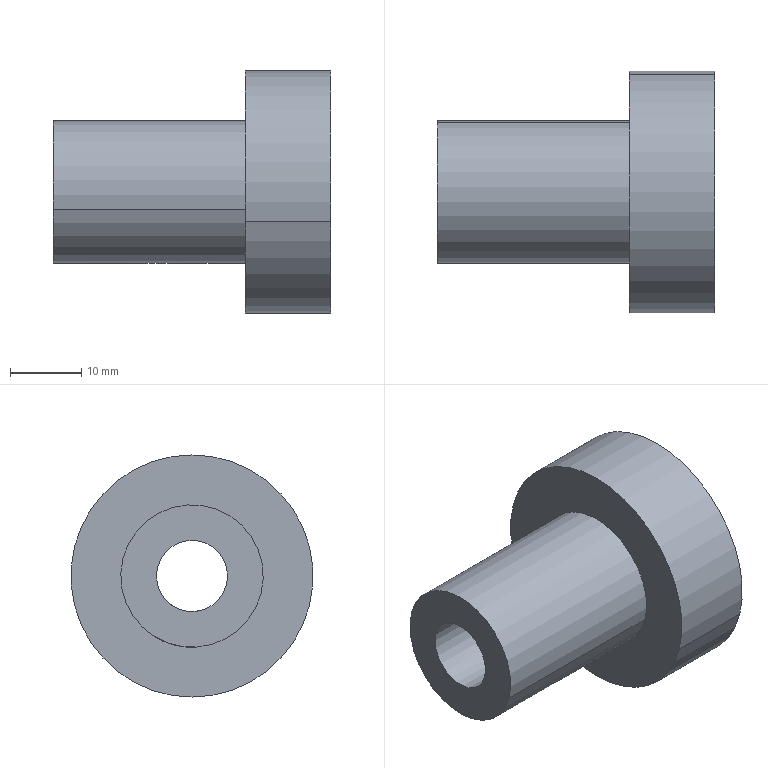Component | SolidWorks | MiddleAxisUpperSleeve-1 | 1 solid | 21 faces | box 39 x 34 x 34 mm | volume 14393 mm3 | cylinder 12 | plane 5 | cone 4 | commonest cylinder face diameters 3.2 x2 17 x2 30 x2 34 x2 20 x2 10 x2 | material 5154-O, Bar (SS)
STEP:
#1=COLOUR_RGB('',0.7922,0.8196,0.9333);
#2=FILL_AREA_STYLE_COLOUR('',#1);
#3=FILL_AREA_STYLE('',(#2));
#4=SURFACE_STYLE_FILL_AREA(#3);
#5=SURFACE_SIDE_STYLE('',(#4));
#6=SURFACE_STYLE_USAGE(.BOTH.,#5);
#7=PRESENTATION_STYLE_ASSIGNMENT((#6));
#8=CARTESIAN_POINT('',(5.711,0.7019,13.575));
#9=VERTEX_POINT('',#8);
#10=CARTESIAN_POINT('',(5.711,0.5797,13.544));
#11=VERTEX_POINT('',#10);
#12=CARTESIAN_POINT('',(5.711,0.7019,13.575));
#13=CARTESIAN_POINT('',(5.719,0.7019,13.575));
#14=CARTESIAN_POINT('',(5.728,0.7004,13.574));
#15=CARTESIAN_POINT('',(5.739,0.6962,13.571));
#16=CARTESIAN_POINT('',(5.743,0.6944,13.57));
#17=CARTESIAN_POINT('',(5.75,0.6903,13.568));
#18=CARTESIAN_POINT('',(5.753,0.6879,13.567));
#19=CARTESIAN_POINT('',(5.761,0.68,13.562));
#20=CARTESIAN_POINT('',(5.766,0.6736,13.559));
#21=CARTESIAN_POINT('',(5.771,0.6628,13.555));
#22=CARTESIAN_POINT('',(5.772,0.6591,13.554));
#23=CARTESIAN_POINT('',(5.774,0.6514,13.551));
#24=CARTESIAN_POINT('',(5.774,0.6474,13.55));
#25=CARTESIAN_POINT('',(5.774,0.6393,13.548));
#26=CARTESIAN_POINT('',(5.774,0.6353,13.547));
#27=CARTESIAN_POINT('',(5.772,0.6273,13.546));
#28=CARTESIAN_POINT('',(5.771,0.6233,13.545));
#29=CARTESIAN_POINT('',(5.766,0.6119,13.544));
#30=CARTESIAN_POINT('',(5.761,0.6048,13.543));
#31=CARTESIAN_POINT('',(5.753,0.596,13.543));
#32=CARTESIAN_POINT('',(5.75,0.5932,13.543));
#33=CARTESIAN_POINT('',(5.743,0.5885,13.543));
#34=CARTESIAN_POINT('',(5.739,0.5865,13.543));
#35=CARTESIAN_POINT('',(5.732,0.5832,13.544));
#36=CARTESIAN_POINT('',(5.728,0.5819,13.544));
#37=CARTESIAN_POINT('',(5.719,0.5802,13.544));
#38=CARTESIAN_POINT('',(5.715,0.5797,13.544));
#39=CARTESIAN_POINT('',(5.711,0.5797,13.544));
#40=B_SPLINE_CURVE_WITH_KNOTS('',3,(#12,#13,#14,#15,#16,#17,#18,#19,#20,#21,#22,#23,#24,#25,#26,#27,#28,#29,#30,#31,#32,#33,#34,#35,#36,#37,#38,#39),.UNSPECIFIED.,.F.,.F.,(4,2,2,2,2,2,2,2,2,2,2,2,2,4),(0.005036,0.005665,0.005979,0.006294,0.006923,0.007238,0.007553,0.007867,0.008182,0.008811,0.009126,0.00944,0.009755,0.01007),.UNSPECIFIED.);
#41=EDGE_CURVE('',#9,#11,#40,.T.);
#42=ORIENTED_EDGE('',*,*,#41,.F.);
#43=CARTESIAN_POINT('',(5.711,0.7372,13.435));
#44=VERTEX_POINT('',#43);
#45=CARTESIAN_POINT('',(5.711,0.7527,13.374));
#46=DIRECTION('',(0.,0.2451,-0.9695));
#47=VECTOR('',#46,39.37);
#48=LINE('',#45,#47);
#49=EDGE_CURVE('',#9,#44,#48,.T.);
#50=ORIENTED_EDGE('',*,*,#49,.T.);
#51=CARTESIAN_POINT('',(5.711,0.6151,13.404));
#52=VERTEX_POINT('',#51);
#53=CARTESIAN_POINT('',(5.711,0.6762,13.42));
#54=DIRECTION('',(0.,0.2451,-0.9695));
#55=DIRECTION('',(0.,-0.9695,-0.2451));
#56=AXIS2_PLACEMENT_3D('',#53,#54,#55);
#57=CIRCLE('',#56,0.06299);
#58=EDGE_CURVE('',#44,#52,#57,.T.);
#59=ORIENTED_EDGE('',*,*,#58,.T.);
#60=CARTESIAN_POINT('',(5.711,0.6305,13.343));
#61=DIRECTION('',(0.,0.2451,-0.9695));
#62=VECTOR('',#61,39.37);
#63=LINE('',#60,#62);
#64=EDGE_CURVE('',#11,#52,#63,.T.);
#65=ORIENTED_EDGE('',*,*,#64,.F.);
#66=EDGE_LOOP('',(#42,#50,#59,#65));
#67=FACE_OUTER_BOUND('',#66,.T.);
#68=CARTESIAN_POINT('',(5.711,0.6916,13.358));
#69=DIRECTION('',(0.,0.2451,-0.9695));
#70=DIRECTION('',(0.,-0.9695,-0.2451));
#71=AXIS2_PLACEMENT_3D('',#68,#69,#70);
#72=CYLINDRICAL_SURFACE('',#71,0.06299);
#73=ADVANCED_FACE('',(#67),#72,.F.);
#74=ORIENTED_EDGE('',*,*,#58,.F.);
#75=CARTESIAN_POINT('',(5.711,0.7946,13.401));
#76=VERTEX_POINT('',#75);
#77=CARTESIAN_POINT('',(5.711,0.8137,13.389));
#78=DIRECTION('',(-0.,0.8589,-0.5122));
#79=VECTOR('',#78,39.37);
#80=LINE('',#77,#79);
#81=EDGE_CURVE('',#44,#76,#80,.T.);
#82=ORIENTED_EDGE('',*,*,#81,.T.);
#83=CARTESIAN_POINT('',(5.711,0.5809,13.347));
#84=VERTEX_POINT('',#83);
#85=CARTESIAN_POINT('',(5.711,0.5809,13.347));
#86=CARTESIAN_POINT('',(5.727,0.5809,13.347));
#87=CARTESIAN_POINT('',(5.742,0.5836,13.347));
#88=CARTESIAN_POINT('',(5.764,0.5913,13.346));
#89=CARTESIAN_POINT('',(5.771,0.5945,13.346));
#90=CARTESIAN_POINT('',(5.785,0.6022,13.347));
#91=CARTESIAN_POINT('',(5.791,0.6066,13.347));
#92=CARTESIAN_POINT('',(5.803,0.6165,13.347));
#93=CARTESIAN_POINT('',(5.808,0.622,13.347));
#94=CARTESIAN_POINT('',(5.818,0.6341,13.348));
#95=CARTESIAN_POINT('',(5.823,0.6406,13.349));
#96=CARTESIAN_POINT('',(5.83,0.6543,13.351));
#97=CARTESIAN_POINT('',(5.832,0.6616,13.352));
#98=CARTESIAN_POINT('',(5.836,0.6764,13.355));
#99=CARTESIAN_POINT('',(5.837,0.6838,13.357));
#100=CARTESIAN_POINT('',(5.837,0.6991,13.36));
#101=CARTESIAN_POINT('',(5.836,0.7065,13.362));
#102=CARTESIAN_POINT('',(5.832,0.7209,13.367));
#103=CARTESIAN_POINT('',(5.83,0.7279,13.369));
#104=CARTESIAN_POINT('',(5.823,0.7408,13.374));
#105=CARTESIAN_POINT('',(5.818,0.7469,13.377));
#106=CARTESIAN_POINT('',(5.808,0.7581,13.382));
#107=CARTESIAN_POINT('',(5.803,0.7631,13.384));
#108=CARTESIAN_POINT('',(5.785,0.7766,13.391));
#109=CARTESIAN_POINT('',(5.771,0.7833,13.394));
#110=CARTESIAN_POINT('',(5.749,0.7901,13.398));
#111=CARTESIAN_POINT('',(5.742,0.7918,13.399));
#112=CARTESIAN_POINT('',(5.727,0.794,13.4));
#113=CARTESIAN_POINT('',(5.719,0.7946,13.401));
#114=CARTESIAN_POINT('',(5.711,0.7946,13.401));
#115=B_SPLINE_CURVE_WITH_KNOTS('',3,(#85,#86,#87,#88,#89,#90,#91,#92,#93,#94,#95,#96,#97,#98,#99,#100,#101,#102,#103,#104,#105,#106,#107,#108,#109,#110,#111,#112,#113,#114),.UNSPECIFIED.,.F.,.F.,(4,2,2,2,2,2,2,2,2,2,2,2,2,2,4),(0.01171,0.01289,0.01348,0.01406,0.01465,0.01524,0.01583,0.01642,0.017,0.01759,0.01818,0.01877,0.01994,0.02053,0.02112),.UNSPECIFIED.);
#116=EDGE_CURVE('',#84,#76,#115,.T.);
#117=ORIENTED_EDGE('',*,*,#116,.F.);
#118=CARTESIAN_POINT('',(5.711,0.5695,13.328));
#119=DIRECTION('',(0.,-0.5122,-0.8589));
#120=VECTOR('',#119,39.37);
#121=LINE('',#118,#120);
#122=EDGE_CURVE('',#52,#84,#121,.T.);
#123=ORIENTED_EDGE('',*,*,#122,.F.);
#124=EDGE_LOOP('',(#74,#82,#117,#123));
#125=FACE_OUTER_BOUND('',#124,.T.);
#126=CARTESIAN_POINT('',(5.711,0.6916,13.358));
#127=DIRECTION('',(0.,0.2451,-0.9695));
#128=DIRECTION('',(0.,-0.9695,-0.2451));
#129=AXIS2_PLACEMENT_3D('',#126,#127,#128);
#130=CONICAL_SURFACE('',#129,0.126,0.7854);
#131=ADVANCED_FACE('',(#125),#130,.F.);
#132=CARTESIAN_POINT('',(6.42,0.9195,13.822));
#133=VERTEX_POINT('',#132);
#134=CARTESIAN_POINT('',(6.42,0.2707,13.658));
#135=VERTEX_POINT('',#134);
#136=CARTESIAN_POINT('',(6.42,0.5951,13.74));
#137=DIRECTION('',(1.,0.,0.));
#138=DIRECTION('',(0.,-0.9695,-0.2451));
#139=AXIS2_PLACEMENT_3D('',#136,#137,#138);
#140=CIRCLE('',#139,0.3346);
#141=EDGE_CURVE('',#133,#135,#140,.T.);
#142=ORIENTED_EDGE('',*,*,#141,.F.);
#143=CARTESIAN_POINT('',(6.577,0.9195,13.822));
#144=VERTEX_POINT('',#143);
#145=CARTESIAN_POINT('',(9.528,0.9195,13.822));
#146=DIRECTION('',(1.,0.,0.));
#147=VECTOR('',#146,39.37);
#148=LINE('',#145,#147);
#149=EDGE_CURVE('',#133,#144,#148,.T.);
#150=ORIENTED_EDGE('',*,*,#149,.T.);
#151=CARTESIAN_POINT('',(6.577,0.2707,13.658));
#152=VERTEX_POINT('',#151);
#153=CARTESIAN_POINT('',(6.577,0.5951,13.74));
#154=DIRECTION('',(1.,0.,0.));
#155=DIRECTION('',(0.,-0.9695,-0.2451));
#156=AXIS2_PLACEMENT_3D('',#153,#154,#155);
#157=CIRCLE('',#156,0.3346);
#158=EDGE_CURVE('',#144,#152,#157,.T.);
#159=ORIENTED_EDGE('',*,*,#158,.T.);
#160=CARTESIAN_POINT('',(9.528,0.2707,13.658));
#161=DIRECTION('',(1.,0.,0.));
#162=VECTOR('',#161,39.37);
#163=LINE('',#160,#162);
#164=EDGE_CURVE('',#135,#152,#163,.T.);
#165=ORIENTED_EDGE('',*,*,#164,.F.);
#166=EDGE_LOOP('',(#142,#150,#159,#165));
#167=FACE_OUTER_BOUND('',#166,.T.);
#168=CARTESIAN_POINT('',(9.528,0.5951,13.74));
#169=DIRECTION('',(1.,0.,0.));
#170=DIRECTION('',(0.,-0.9695,-0.2451));
#171=AXIS2_PLACEMENT_3D('',#168,#169,#170);
#172=CYLINDRICAL_SURFACE('',#171,0.3346);
#173=ADVANCED_FACE('',(#167),#172,.F.);
#174=CARTESIAN_POINT('',(6.577,1.168,13.885));
#175=VERTEX_POINT('',#174);
#176=CARTESIAN_POINT('',(6.577,0.02257,13.595));
#177=VERTEX_POINT('',#176);
#178=CARTESIAN_POINT('',(6.577,0.5951,13.74));
#179=DIRECTION('',(1.,0.,0.));
#180=DIRECTION('',(0.,-0.9695,-0.2451));
#181=AXIS2_PLACEMENT_3D('',#178,#179,#180);
#182=CIRCLE('',#181,0.5906);
#183=EDGE_CURVE('',#175,#177,#182,.T.);
#184=ORIENTED_EDGE('',*,*,#183,.F.);
#185=CARTESIAN_POINT('',(6.656,1.168,13.885));
#186=VERTEX_POINT('',#185);
#187=CARTESIAN_POINT('',(9.528,1.168,13.885));
#188=DIRECTION('',(1.,0.,0.));
#189=VECTOR('',#188,39.37);
#190=LINE('',#187,#189);
#191=EDGE_CURVE('',#175,#186,#190,.T.);
#192=ORIENTED_EDGE('',*,*,#191,.T.);
#193=CARTESIAN_POINT('',(6.656,0.02257,13.595));
#194=VERTEX_POINT('',#193);
#195=CARTESIAN_POINT('',(6.656,0.5951,13.74));
#196=DIRECTION('',(1.,0.,0.));
#197=DIRECTION('',(0.,-0.9695,-0.2451));
#198=AXIS2_PLACEMENT_3D('',#195,#196,#197);
#199=CIRCLE('',#198,0.5906);
#200=EDGE_CURVE('',#186,#194,#199,.T.);
#201=ORIENTED_EDGE('',*,*,#200,.T.);
#202=CARTESIAN_POINT('',(9.528,0.02257,13.595));
#203=DIRECTION('',(1.,0.,0.));
#204=VECTOR('',#203,39.37);
#205=LINE('',#202,#204);
#206=EDGE_CURVE('',#177,#194,#205,.T.);
#207=ORIENTED_EDGE('',*,*,#206,.F.);
#208=EDGE_LOOP('',(#184,#192,#201,#207));
#209=FACE_OUTER_BOUND('',#208,.T.);
#210=CARTESIAN_POINT('',(9.528,0.5951,13.74));
#211=DIRECTION('',(1.,0.,0.));
#212=DIRECTION('',(0.,-0.9695,-0.2451));
#213=AXIS2_PLACEMENT_3D('',#210,#211,#212);
#214=CYLINDRICAL_SURFACE('',#213,0.5906);
#215=ADVANCED_FACE('',(#209),#214,.F.);
#216=CARTESIAN_POINT('',(6.184,-0.05377,13.576));
#217=VERTEX_POINT('',#216);
#218=CARTESIAN_POINT('',(6.184,1.244,13.904));
#219=VERTEX_POINT('',#218);
#220=CARTESIAN_POINT('',(6.184,0.5951,13.74));
#221=DIRECTION('',(1.,0.,0.));
#222=DIRECTION('',(0.,-0.9695,-0.2451));
#223=AXIS2_PLACEMENT_3D('',#220,#221,#222);
#224=CIRCLE('',#223,0.6693);
#225=EDGE_CURVE('',#217,#219,#224,.T.);
#226=ORIENTED_EDGE('',*,*,#225,.T.);
#227=CARTESIAN_POINT('',(6.656,1.244,13.904));
#228=VERTEX_POINT('',#227);
#229=CARTESIAN_POINT('',(9.528,1.244,13.904));
#230=DIRECTION('',(1.,0.,0.));
#231=VECTOR('',#230,39.37);
#232=LINE('',#229,#231);
#233=EDGE_CURVE('',#219,#228,#232,.T.);
#234=ORIENTED_EDGE('',*,*,#233,.T.);
#235=CARTESIAN_POINT('',(6.656,-0.05377,13.576));
#236=VERTEX_POINT('',#235);
#237=CARTESIAN_POINT('',(6.656,0.5951,13.74));
#238=DIRECTION('',(1.,0.,0.));
#239=DIRECTION('',(0.,-0.9695,-0.2451));
#240=AXIS2_PLACEMENT_3D('',#237,#238,#239);
#241=CIRCLE('',#240,0.6693);
#242=EDGE_CURVE('',#236,#228,#241,.T.);
#243=ORIENTED_EDGE('',*,*,#242,.F.);
#244=CARTESIAN_POINT('',(9.528,-0.05377,13.576));
#245=DIRECTION('',(1.,0.,0.));
#246=VECTOR('',#245,39.37);
#247=LINE('',#244,#246);
#248=EDGE_CURVE('',#217,#236,#247,.T.);
#249=ORIENTED_EDGE('',*,*,#248,.F.);
#250=EDGE_LOOP('',(#226,#234,#243,#249));
#251=FACE_OUTER_BOUND('',#250,.T.);
#252=CARTESIAN_POINT('',(9.528,0.5951,13.74));
#253=DIRECTION('',(1.,0.,0.));
#254=DIRECTION('',(0.,-0.9695,-0.2451));
#255=AXIS2_PLACEMENT_3D('',#252,#253,#254);
#256=CYLINDRICAL_SURFACE('',#255,0.6693);
#257=ADVANCED_FACE('',(#251),#256,.T.);
#258=ORIENTED_EDGE('',*,*,#116,.T.);
#259=CARTESIAN_POINT('',(5.711,0.7946,13.401));
#260=CARTESIAN_POINT('',(5.703,0.7946,13.401));
#261=CARTESIAN_POINT('',(5.696,0.794,13.4));
#262=CARTESIAN_POINT('',(5.68,0.7918,13.399));
#263=CARTESIAN_POINT('',(5.673,0.7901,13.398));
#264=CARTESIAN_POINT('',(5.658,0.7855,13.396));
#265=CARTESIAN_POINT('',(5.651,0.7827,13.394));
#266=CARTESIAN_POINT('',(5.638,0.776,13.39));
#267=CARTESIAN_POINT('',(5.631,0.7721,13.388));
#268=CARTESIAN_POINT('',(5.619,0.7631,13.384));
#269=CARTESIAN_POINT('',(5.614,0.7581,13.382));
#270=CARTESIAN_POINT('',(5.604,0.7472,13.377));
#271=CARTESIAN_POINT('',(5.6,0.7411,13.374));
#272=CARTESIAN_POINT('',(5.593,0.7282,13.37));
#273=CARTESIAN_POINT('',(5.59,0.7214,13.367));
#274=CARTESIAN_POINT('',(5.586,0.7071,13.363));
#275=CARTESIAN_POINT('',(5.585,0.6995,13.36));
#276=CARTESIAN_POINT('',(5.585,0.6845,13.357));
#277=CARTESIAN_POINT('',(5.586,0.6769,13.355));
#278=CARTESIAN_POINT('',(5.59,0.6619,13.352));
#279=CARTESIAN_POINT('',(5.592,0.6548,13.351));
#280=CARTESIAN_POINT('',(5.603,0.634,13.348));
#281=CARTESIAN_POINT('',(5.613,0.6217,13.347));
#282=CARTESIAN_POINT('',(5.631,0.6067,13.347));
#283=CARTESIAN_POINT('',(5.637,0.6023,13.347));
#284=CARTESIAN_POINT('',(5.651,0.5946,13.346));
#285=CARTESIAN_POINT('',(5.658,0.5914,13.346));
#286=CARTESIAN_POINT('',(5.673,0.5862,13.347));
#287=CARTESIAN_POINT('',(5.68,0.5842,13.347));
#288=CARTESIAN_POINT('',(5.696,0.5815,13.347));
#289=CARTESIAN_POINT('',(5.703,0.5809,13.347));
#290=CARTESIAN_POINT('',(5.711,0.5809,13.347));
#291=B_SPLINE_CURVE_WITH_KNOTS('',3,(#259,#260,#261,#262,#263,#264,#265,#266,#267,#268,#269,#270,#271,#272,#273,#274,#275,#276,#277,#278,#279,#280,#281,#282,#283,#284,#285,#286,#287,#288,#289,#290),.UNSPECIFIED.,.F.,.F.,(4,2,2,2,2,2,2,2,2,2,2,2,2,2,2,4),(0.0023,0.002888,0.003477,0.004065,0.004653,0.005242,0.00583,0.006419,0.007007,0.007595,0.008184,0.00936,0.009949,0.01054,0.01113,0.01171),.UNSPECIFIED.);
#292=EDGE_CURVE('',#76,#84,#291,.T.);
#293=ORIENTED_EDGE('',*,*,#292,.T.);
#294=EDGE_LOOP('',(#258,#293));
#295=FACE_BOUND('',#294,.T.);
#296=CARTESIAN_POINT('',(5.121,0.2134,13.644));
#297=VERTEX_POINT('',#296);
#298=CARTESIAN_POINT('',(5.121,0.9768,13.837));
#299=VERTEX_POINT('',#298);
#300=CARTESIAN_POINT('',(5.121,0.5951,13.74));
#301=DIRECTION('',(1.,0.,0.));
#302=DIRECTION('',(0.,-0.9695,-0.2451));
#303=AXIS2_PLACEMENT_3D('',#300,#301,#302);
#304=CIRCLE('',#303,0.3937);
#305=EDGE_CURVE('',#297,#299,#304,.T.);
#306=ORIENTED_EDGE('',*,*,#305,.T.);
#307=CARTESIAN_POINT('',(6.184,0.9768,13.837));
#308=VERTEX_POINT('',#307);
#309=CARTESIAN_POINT('',(9.528,0.9768,13.837));
#310=DIRECTION('',(1.,0.,0.));
#311=VECTOR('',#310,39.37);
#312=LINE('',#309,#311);
#313=EDGE_CURVE('',#299,#308,#312,.T.);
#314=ORIENTED_EDGE('',*,*,#313,.T.);
#315=CARTESIAN_POINT('',(6.184,0.2134,13.644));
#316=VERTEX_POINT('',#315);
#317=CARTESIAN_POINT('',(6.184,0.5951,13.74));
#318=DIRECTION('',(1.,0.,0.));
#319=DIRECTION('',(0.,-0.9695,-0.2451));
#320=AXIS2_PLACEMENT_3D('',#317,#318,#319);
#321=CIRCLE('',#320,0.3937);
#322=EDGE_CURVE('',#316,#308,#321,.T.);
#323=ORIENTED_EDGE('',*,*,#322,.F.);
#324=CARTESIAN_POINT('',(9.528,0.2134,13.644));
#325=DIRECTION('',(1.,0.,0.));
#326=VECTOR('',#325,39.37);
#327=LINE('',#324,#326);
#328=EDGE_CURVE('',#297,#316,#327,.T.);
#329=ORIENTED_EDGE('',*,*,#328,.F.);
#330=EDGE_LOOP('',(#306,#314,#323,#329));
#331=FACE_OUTER_BOUND('',#330,.T.);
#332=CARTESIAN_POINT('',(9.528,0.5951,13.74));
#333=DIRECTION('',(1.,0.,0.));
#334=DIRECTION('',(0.,-0.9695,-0.2451));
#335=AXIS2_PLACEMENT_3D('',#332,#333,#334);
#336=CYLINDRICAL_SURFACE('',#335,0.3937);
#337=ADVANCED_FACE('',(#295,#331),#336,.T.);
#338=CARTESIAN_POINT('',(5.121,0.786,13.788));
#339=VERTEX_POINT('',#338);
#340=CARTESIAN_POINT('',(5.121,0.4043,13.692));
#341=VERTEX_POINT('',#340);
#342=CARTESIAN_POINT('',(5.121,0.5951,13.74));
#343=DIRECTION('',(1.,0.,0.));
#344=DIRECTION('',(0.,-0.9695,-0.2451));
#345=AXIS2_PLACEMENT_3D('',#342,#343,#344);
#346=CIRCLE('',#345,0.1969);
#347=EDGE_CURVE('',#339,#341,#346,.T.);
#348=ORIENTED_EDGE('',*,*,#347,.F.);
#349=CARTESIAN_POINT('',(6.38,0.786,13.788));
#350=VERTEX_POINT('',#349);
#351=CARTESIAN_POINT('',(9.528,0.786,13.788));
#352=DIRECTION('',(1.,0.,0.));
#353=VECTOR('',#352,39.37);
#354=LINE('',#351,#353);
#355=EDGE_CURVE('',#339,#350,#354,.T.);
#356=ORIENTED_EDGE('',*,*,#355,.T.);
#357=CARTESIAN_POINT('',(6.38,0.4043,13.692));
#358=VERTEX_POINT('',#357);
#359=CARTESIAN_POINT('',(6.38,0.5951,13.74));
#360=DIRECTION('',(1.,0.,0.));
#361=DIRECTION('',(0.,-0.9695,-0.2451));
#362=AXIS2_PLACEMENT_3D('',#359,#360,#361);
#363=CIRCLE('',#362,0.1969);
#364=EDGE_CURVE('',#350,#358,#363,.T.);
#365=ORIENTED_EDGE('',*,*,#364,.T.);
#366=CARTESIAN_POINT('',(9.528,0.4043,13.692));
#367=DIRECTION('',(1.,0.,0.));
#368=VECTOR('',#367,39.37);
#369=LINE('',#366,#368);
#370=EDGE_CURVE('',#341,#358,#369,.T.);
#371=ORIENTED_EDGE('',*,*,#370,.F.);
#372=EDGE_LOOP('',(#348,#356,#365,#371));
#373=FACE_OUTER_BOUND('',#372,.T.);
#374=CARTESIAN_POINT('',(9.528,0.5951,13.74));
#375=DIRECTION('',(1.,0.,0.));
#376=DIRECTION('',(0.,-0.9695,-0.2451));
#377=AXIS2_PLACEMENT_3D('',#374,#375,#376);
#378=CYLINDRICAL_SURFACE('',#377,0.1969);
#379=ADVANCED_FACE('',(#373),#378,.F.);
#380=ORIENTED_EDGE('',*,*,#364,.F.);
#381=CARTESIAN_POINT('',(6.42,0.8241,13.798));
#382=VERTEX_POINT('',#381);
#383=CARTESIAN_POINT('',(6.42,0.8241,13.798));
#384=DIRECTION('',(0.7071,0.6855,0.1733));
#385=VECTOR('',#384,39.37);
#386=LINE('',#383,#385);
#387=EDGE_CURVE('',#350,#382,#386,.T.);
#388=ORIENTED_EDGE('',*,*,#387,.T.);
#389=CARTESIAN_POINT('',(6.42,0.3661,13.682));
#390=VERTEX_POINT('',#389);
#391=CARTESIAN_POINT('',(6.42,0.5951,13.74));
#392=DIRECTION('',(1.,0.,0.));
#393=DIRECTION('',(0.,-0.9695,-0.2451));
#394=AXIS2_PLACEMENT_3D('',#391,#392,#393);
#395=CIRCLE('',#394,0.2362);
#396=EDGE_CURVE('',#382,#390,#395,.T.);
#397=ORIENTED_EDGE('',*,*,#396,.T.);
#398=CARTESIAN_POINT('',(6.42,0.3661,13.682));
#399=DIRECTION('',(0.7071,-0.6855,-0.1733));
#400=VECTOR('',#399,39.37);
#401=LINE('',#398,#400);
#402=EDGE_CURVE('',#358,#390,#401,.T.);
#403=ORIENTED_EDGE('',*,*,#402,.F.);
#404=EDGE_LOOP('',(#380,#388,#397,#403));
#405=FACE_OUTER_BOUND('',#404,.T.);
#406=CARTESIAN_POINT('',(6.42,0.5951,13.74));
#407=DIRECTION('',(1.,0.,0.));
#408=DIRECTION('',(0.,-0.9695,-0.2451));
#409=AXIS2_PLACEMENT_3D('',#406,#407,#408);
#410=CONICAL_SURFACE('',#409,0.2362,0.7854);
#411=ADVANCED_FACE('',(#405),#410,.F.);
#412=ORIENTED_EDGE('',*,*,#387,.F.);
#413=CARTESIAN_POINT('',(6.38,0.5951,13.74));
#414=DIRECTION('',(1.,0.,0.));
#415=DIRECTION('',(0.,-0.9695,-0.2451));
#416=AXIS2_PLACEMENT_3D('',#413,#414,#415);
#417=CIRCLE('',#416,0.1969);
#418=EDGE_CURVE('',#358,#350,#417,.T.);
#419=ORIENTED_EDGE('',*,*,#418,.F.);
#420=ORIENTED_EDGE('',*,*,#402,.T.);
#421=CARTESIAN_POINT('',(6.42,0.5951,13.74));
#422=DIRECTION('',(1.,0.,0.));
#423=DIRECTION('',(0.,-0.9695,-0.2451));
#424=AXIS2_PLACEMENT_3D('',#421,#422,#423);
#425=CIRCLE('',#424,0.2362);
#426=EDGE_CURVE('',#390,#382,#425,.T.);
#427=ORIENTED_EDGE('',*,*,#426,.T.);
#428=EDGE_LOOP('',(#412,#419,#420,#427));
#429=FACE_OUTER_BOUND('',#428,.T.);
#430=CARTESIAN_POINT('',(6.42,0.5951,13.74));
#431=DIRECTION('',(1.,0.,0.));
#432=DIRECTION('',(0.,-0.9695,-0.2451));
#433=AXIS2_PLACEMENT_3D('',#430,#431,#432);
#434=CONICAL_SURFACE('',#433,0.2362,0.7854);
#435=ADVANCED_FACE('',(#429),#434,.F.);
#436=ORIENTED_EDGE('',*,*,#355,.F.);
#437=CARTESIAN_POINT('',(5.121,0.5951,13.74));
#438=DIRECTION('',(1.,0.,0.));
#439=DIRECTION('',(0.,-0.9695,-0.2451));
#440=AXIS2_PLACEMENT_3D('',#437,#438,#439);
#441=CIRCLE('',#440,0.1969);
#442=EDGE_CURVE('',#341,#339,#441,.T.);
#443=ORIENTED_EDGE('',*,*,#442,.F.);
#444=ORIENTED_EDGE('',*,*,#370,.T.);
#445=ORIENTED_EDGE('',*,*,#418,.T.);
#446=EDGE_LOOP('',(#436,#443,#444,#445));
#447=FACE_OUTER_BOUND('',#446,.T.);
#448=CARTESIAN_POINT('',(5.711,0.5797,13.544));
#449=CARTESIAN_POINT('',(5.707,0.5797,13.544));
#450=CARTESIAN_POINT('',(5.703,0.5802,13.544));
#451=CARTESIAN_POINT('',(5.695,0.5819,13.544));
#452=CARTESIAN_POINT('',(5.691,0.5832,13.544));
#453=CARTESIAN_POINT('',(5.683,0.5865,13.543));
#454=CARTESIAN_POINT('',(5.679,0.5885,13.543));
#455=CARTESIAN_POINT('',(5.673,0.5932,13.543));
#456=CARTESIAN_POINT('',(5.669,0.596,13.543));
#457=CARTESIAN_POINT('',(5.661,0.6049,13.543));
#458=CARTESIAN_POINT('',(5.656,0.6119,13.544));
#459=CARTESIAN_POINT('',(5.651,0.6233,13.545));
#460=CARTESIAN_POINT('',(5.65,0.6273,13.546));
#461=CARTESIAN_POINT('',(5.649,0.6353,13.547));
#462=CARTESIAN_POINT('',(5.648,0.6393,13.548));
#463=CARTESIAN_POINT('',(5.648,0.6473,13.55));
#464=CARTESIAN_POINT('',(5.649,0.6514,13.551));
#465=CARTESIAN_POINT('',(5.65,0.6591,13.554));
#466=CARTESIAN_POINT('',(5.651,0.6628,13.555));
#467=CARTESIAN_POINT('',(5.656,0.6736,13.559));
#468=CARTESIAN_POINT('',(5.661,0.68,13.562));
#469=CARTESIAN_POINT('',(5.669,0.688,13.567));
#470=CARTESIAN_POINT('',(5.673,0.6903,13.568));
#471=CARTESIAN_POINT('',(5.679,0.6944,13.57));
#472=CARTESIAN_POINT('',(5.683,0.6962,13.571));
#473=CARTESIAN_POINT('',(5.691,0.699,13.573));
#474=CARTESIAN_POINT('',(5.695,0.7001,13.574));
#475=CARTESIAN_POINT('',(5.703,0.7015,13.575));
#476=CARTESIAN_POINT('',(5.707,0.7019,13.575));
#477=CARTESIAN_POINT('',(5.711,0.7019,13.575));
#478=B_SPLINE_CURVE_WITH_KNOTS('',3,(#448,#449,#450,#451,#452,#453,#454,#455,#456,#457,#458,#459,#460,#461,#462,#463,#464,#465,#466,#467,#468,#469,#470,#471,#472,#473,#474,#475,#476,#477),.UNSPECIFIED.,.F.,.F.,(4,2,2,2,2,2,2,2,2,2,2,2,2,2,4),(0.,0.0003147,0.0006294,0.0009442,0.001259,0.001888,0.002203,0.002518,0.002833,0.003147,0.003777,0.004091,0.004406,0.004721,0.005036),.UNSPECIFIED.);
#479=EDGE_CURVE('',#11,#9,#478,.T.);
#480=ORIENTED_EDGE('',*,*,#479,.T.);
#481=ORIENTED_EDGE('',*,*,#41,.T.);
#482=EDGE_LOOP('',(#480,#481));
#483=FACE_BOUND('',#482,.T.);
#484=CARTESIAN_POINT('',(9.528,0.5951,13.74));
#485=DIRECTION('',(1.,0.,0.));
#486=DIRECTION('',(0.,-0.9695,-0.2451));
#487=AXIS2_PLACEMENT_3D('',#484,#485,#486);
#488=CYLINDRICAL_SURFACE('',#487,0.1969);
#489=ADVANCED_FACE('',(#447,#483),#488,.F.);
#490=ORIENTED_EDGE('',*,*,#305,.F.);
#491=CARTESIAN_POINT('',(5.121,0.5951,13.74));
#492=DIRECTION('',(1.,0.,0.));
#493=DIRECTION('',(0.,-0.9695,-0.2451));
#494=AXIS2_PLACEMENT_3D('',#491,#492,#493);
#495=CIRCLE('',#494,0.3937);
#496=EDGE_CURVE('',#299,#297,#495,.T.);
#497=ORIENTED_EDGE('',*,*,#496,.F.);
#498=EDGE_LOOP('',(#490,#497));
#499=FACE_OUTER_BOUND('',#498,.T.);
#500=ORIENTED_EDGE('',*,*,#442,.T.);
#501=ORIENTED_EDGE('',*,*,#347,.T.);
#502=EDGE_LOOP('',(#500,#501));
#503=FACE_BOUND('',#502,.T.);
#504=CARTESIAN_POINT('',(5.121,0.6916,13.358));
#505=DIRECTION('',(1.,0.,0.));
#506=DIRECTION('',(0.,-0.9695,-0.2451));
#507=AXIS2_PLACEMENT_3D('',#504,#505,#506);
#508=PLANE('',#507);
#509=ADVANCED_FACE('',(#499,#503),#508,.F.);
#510=ORIENTED_EDGE('',*,*,#313,.F.);
#511=ORIENTED_EDGE('',*,*,#496,.T.);
#512=ORIENTED_EDGE('',*,*,#328,.T.);
#513=CARTESIAN_POINT('',(6.184,0.5951,13.74));
#514=DIRECTION('',(1.,0.,0.));
#515=DIRECTION('',(0.,-0.9695,-0.2451));
#516=AXIS2_PLACEMENT_3D('',#513,#514,#515);
#517=CIRCLE('',#516,0.3937);
#518=EDGE_CURVE('',#308,#316,#517,.T.);
#519=ORIENTED_EDGE('',*,*,#518,.F.);
#520=EDGE_LOOP('',(#510,#511,#512,#519));
#521=FACE_OUTER_BOUND('',#520,.T.);
#522=CARTESIAN_POINT('',(9.528,0.5951,13.74));
#523=DIRECTION('',(1.,0.,0.));
#524=DIRECTION('',(0.,-0.9695,-0.2451));
#525=AXIS2_PLACEMENT_3D('',#522,#523,#524);
#526=CYLINDRICAL_SURFACE('',#525,0.3937);
#527=ADVANCED_FACE('',(#521),#526,.T.);
#528=ORIENTED_EDGE('',*,*,#225,.F.);
#529=CARTESIAN_POINT('',(6.184,0.5951,13.74));
#530=DIRECTION('',(1.,0.,0.));
#531=DIRECTION('',(0.,-0.9695,-0.2451));
#532=AXIS2_PLACEMENT_3D('',#529,#530,#531);
#533=CIRCLE('',#532,0.6693);
#534=EDGE_CURVE('',#219,#217,#533,.T.);
#535=ORIENTED_EDGE('',*,*,#534,.F.);
#536=EDGE_LOOP('',(#528,#535));
#537=FACE_OUTER_BOUND('',#536,.T.);
#538=ORIENTED_EDGE('',*,*,#322,.T.);
#539=ORIENTED_EDGE('',*,*,#518,.T.);
#540=EDGE_LOOP('',(#538,#539));
#541=FACE_BOUND('',#540,.T.);
#542=CARTESIAN_POINT('',(6.184,0.7592,13.091));
#543=DIRECTION('',(1.,0.,0.));
#544=DIRECTION('',(0.,-0.9695,-0.2451));
#545=AXIS2_PLACEMENT_3D('',#542,#543,#544);
#546=PLANE('',#545);
#547=ADVANCED_FACE('',(#537,#541),#546,.F.);
#548=ORIENTED_EDGE('',*,*,#233,.F.);
#549=ORIENTED_EDGE('',*,*,#534,.T.);
#550=ORIENTED_EDGE('',*,*,#248,.T.);
#551=CARTESIAN_POINT('',(6.656,0.5951,13.74));
#552=DIRECTION('',(1.,0.,0.));
#553=DIRECTION('',(0.,-0.9695,-0.2451));
#554=AXIS2_PLACEMENT_3D('',#551,#552,#553);
#555=CIRCLE('',#554,0.6693);
#556=EDGE_CURVE('',#228,#236,#555,.T.);
#557=ORIENTED_EDGE('',*,*,#556,.F.);
#558=EDGE_LOOP('',(#548,#549,#550,#557));
#559=FACE_OUTER_BOUND('',#558,.T.);
#560=CARTESIAN_POINT('',(9.528,0.5951,13.74));
#561=DIRECTION('',(1.,0.,0.));
#562=DIRECTION('',(0.,-0.9695,-0.2451));
#563=AXIS2_PLACEMENT_3D('',#560,#561,#562);
#564=CYLINDRICAL_SURFACE('',#563,0.6693);
#565=ADVANCED_FACE('',(#559),#564,.T.);
#566=CARTESIAN_POINT('',(6.656,0.5951,13.74));
#567=DIRECTION('',(1.,0.,0.));
#568=DIRECTION('',(0.,-0.9695,-0.2451));
#569=AXIS2_PLACEMENT_3D('',#566,#567,#568);
#570=CIRCLE('',#569,0.5906);
#571=EDGE_CURVE('',#194,#186,#570,.T.);
#572=ORIENTED_EDGE('',*,*,#571,.F.);
#573=ORIENTED_EDGE('',*,*,#200,.F.);
#574=EDGE_LOOP('',(#572,#573));
#575=FACE_BOUND('',#574,.T.);
#576=ORIENTED_EDGE('',*,*,#242,.T.);
#577=ORIENTED_EDGE('',*,*,#556,.T.);
#578=EDGE_LOOP('',(#576,#577));
#579=FACE_OUTER_BOUND('',#578,.T.);
#580=CARTESIAN_POINT('',(6.656,0.7399,13.168));
#581=DIRECTION('',(-1.,0.,0.));
#582=DIRECTION('',(0.,0.9695,0.2451));
#583=AXIS2_PLACEMENT_3D('',#580,#581,#582);
#584=PLANE('',#583);
#585=ADVANCED_FACE('',(#575,#579),#584,.F.);
#586=ORIENTED_EDGE('',*,*,#191,.F.);
#587=CARTESIAN_POINT('',(6.577,0.5951,13.74));
#588=DIRECTION('',(1.,0.,0.));
#589=DIRECTION('',(0.,-0.9695,-0.2451));
#590=AXIS2_PLACEMENT_3D('',#587,#588,#589);
#591=CIRCLE('',#590,0.5906);
#592=EDGE_CURVE('',#177,#175,#591,.T.);
#593=ORIENTED_EDGE('',*,*,#592,.F.);
#594=ORIENTED_EDGE('',*,*,#206,.T.);
#595=ORIENTED_EDGE('',*,*,#571,.T.);
#596=EDGE_LOOP('',(#586,#593,#594,#595));
#597=FACE_OUTER_BOUND('',#596,.T.);
#598=CARTESIAN_POINT('',(9.528,0.5951,13.74));
#599=DIRECTION('',(1.,0.,0.));
#600=DIRECTION('',(0.,-0.9695,-0.2451));
#601=AXIS2_PLACEMENT_3D('',#598,#599,#600);
#602=CYLINDRICAL_SURFACE('',#601,0.5906);
#603=ADVANCED_FACE('',(#597),#602,.F.);
#604=CARTESIAN_POINT('',(6.577,0.5951,13.74));
#605=DIRECTION('',(1.,0.,0.));
#606=DIRECTION('',(0.,-0.9695,-0.2451));
#607=AXIS2_PLACEMENT_3D('',#604,#605,#606);
#608=CIRCLE('',#607,0.3346);
#609=EDGE_CURVE('',#152,#144,#608,.T.);
#610=ORIENTED_EDGE('',*,*,#609,.F.);
#611=ORIENTED_EDGE('',*,*,#158,.F.);
#612=EDGE_LOOP('',(#610,#611));
#613=FACE_BOUND('',#612,.T.);
#614=ORIENTED_EDGE('',*,*,#592,.T.);
#615=ORIENTED_EDGE('',*,*,#183,.T.);
#616=EDGE_LOOP('',(#614,#615));
#617=FACE_OUTER_BOUND('',#616,.T.);
#618=CARTESIAN_POINT('',(6.577,0.7399,13.168));
#619=DIRECTION('',(-1.,0.,0.));
#620=DIRECTION('',(0.,0.9695,0.2451));
#621=AXIS2_PLACEMENT_3D('',#618,#619,#620);
#622=PLANE('',#621);
#623=ADVANCED_FACE('',(#613,#617),#622,.F.);
#624=ORIENTED_EDGE('',*,*,#149,.F.);
#625=CARTESIAN_POINT('',(6.42,0.5951,13.74));
#626=DIRECTION('',(1.,0.,0.));
#627=DIRECTION('',(0.,-0.9695,-0.2451));
#628=AXIS2_PLACEMENT_3D('',#625,#626,#627);
#629=CIRCLE('',#628,0.3346);
#630=EDGE_CURVE('',#135,#133,#629,.T.);
#631=ORIENTED_EDGE('',*,*,#630,.F.);
#632=ORIENTED_EDGE('',*,*,#164,.T.);
#633=ORIENTED_EDGE('',*,*,#609,.T.);
#634=EDGE_LOOP('',(#624,#631,#632,#633));
#635=FACE_OUTER_BOUND('',#634,.T.);
#636=CARTESIAN_POINT('',(9.528,0.5951,13.74));
#637=DIRECTION('',(1.,0.,0.));
#638=DIRECTION('',(0.,-0.9695,-0.2451));
#639=AXIS2_PLACEMENT_3D('',#636,#637,#638);
#640=CYLINDRICAL_SURFACE('',#639,0.3346);
#641=ADVANCED_FACE('',(#635),#640,.F.);
#642=ORIENTED_EDGE('',*,*,#426,.F.);
#643=ORIENTED_EDGE('',*,*,#396,.F.);
#644=EDGE_LOOP('',(#642,#643));
#645=FACE_BOUND('',#644,.T.);
#646=ORIENTED_EDGE('',*,*,#630,.T.);
#647=ORIENTED_EDGE('',*,*,#141,.T.);
#648=EDGE_LOOP('',(#646,#647));
#649=FACE_OUTER_BOUND('',#648,.T.);
#650=CARTESIAN_POINT('',(6.42,0.6771,13.416));
#651=DIRECTION('',(-1.,0.,0.));
#652=DIRECTION('',(0.,0.9695,0.2451));
#653=AXIS2_PLACEMENT_3D('',#650,#651,#652);
#654=PLANE('',#653);
#655=ADVANCED_FACE('',(#645,#649),#654,.F.);
#656=ORIENTED_EDGE('',*,*,#81,.F.);
#657=CARTESIAN_POINT('',(5.711,0.6762,13.42));
#658=DIRECTION('',(0.,0.2451,-0.9695));
#659=DIRECTION('',(0.,-0.9695,-0.2451));
#660=AXIS2_PLACEMENT_3D('',#657,#658,#659);
#661=CIRCLE('',#660,0.06299);
#662=EDGE_CURVE('',#52,#44,#661,.T.);
#663=ORIENTED_EDGE('',*,*,#662,.F.);
#664=ORIENTED_EDGE('',*,*,#122,.T.);
#665=ORIENTED_EDGE('',*,*,#292,.F.);
#666=EDGE_LOOP('',(#656,#663,#664,#665));
#667=FACE_OUTER_BOUND('',#666,.T.);
#668=CARTESIAN_POINT('',(5.711,0.6916,13.358));
#669=DIRECTION('',(0.,0.2451,-0.9695));
#670=DIRECTION('',(0.,-0.9695,-0.2451));
#671=AXIS2_PLACEMENT_3D('',#668,#669,#670);
#672=CONICAL_SURFACE('',#671,0.126,0.7854);
#673=ADVANCED_FACE('',(#667),#672,.F.);
#674=ORIENTED_EDGE('',*,*,#49,.F.);
#675=ORIENTED_EDGE('',*,*,#479,.F.);
#676=ORIENTED_EDGE('',*,*,#64,.T.);
#677=ORIENTED_EDGE('',*,*,#662,.T.);
#678=EDGE_LOOP('',(#674,#675,#676,#677));
#679=FACE_OUTER_BOUND('',#678,.T.);
#680=CARTESIAN_POINT('',(5.711,0.6916,13.358));
#681=DIRECTION('',(0.,0.2451,-0.9695));
#682=DIRECTION('',(0.,-0.9695,-0.2451));
#683=AXIS2_PLACEMENT_3D('',#680,#681,#682);
#684=CYLINDRICAL_SURFACE('',#683,0.06299);
#685=ADVANCED_FACE('',(#679),#684,.F.);
#686=CLOSED_SHELL('',(#73,#131,#173,#215,#257,#337,#379,#411,#435,#489,#509,#527,#547,#565,#585,#603,#623,#641,#655,#673,#685));
#687=MANIFOLD_SOLID_BREP('',#686);
#688=STYLED_ITEM('',(#7),#687);
#689=(LENGTH_UNIT()NAMED_UNIT(*)SI_UNIT($,.METRE.));
#690=LENGTH_MEASURE_WITH_UNIT(LENGTH_MEASURE(0.0254),#689);
#691=DIMENSIONAL_EXPONENTS(1.,0.,0.,0.,0.,0.,0.);
#692=(CONVERSION_BASED_UNIT('',#690)LENGTH_UNIT()NAMED_UNIT(#691));
#693=UNCERTAINTY_MEASURE_WITH_UNIT(LENGTH_MEASURE(0.00001),#692,'','');
#694=(NAMED_UNIT(*)PLANE_ANGLE_UNIT()SI_UNIT($,.RADIAN.));
#695=(NAMED_UNIT(*)SI_UNIT($,.STERADIAN.)SOLID_ANGLE_UNIT());
#696=(GEOMETRIC_REPRESENTATION_CONTEXT(3)GLOBAL_UNCERTAINTY_ASSIGNED_CONTEXT((#693))GLOBAL_UNIT_ASSIGNED_CONTEXT((#692,#694,#695))REPRESENTATION_CONTEXT('',''));
#697=MECHANICAL_DESIGN_GEOMETRIC_PRESENTATION_REPRESENTATION('',(#688),#696);
#698=CARTESIAN_POINT('',(0.,0.,0.));
#699=DIRECTION('',(0.,0.,1.));
#700=DIRECTION('',(1.,0.,0.));
#701=AXIS2_PLACEMENT_3D('',#698,#699,#700);
#702=(LENGTH_UNIT()NAMED_UNIT(*)SI_UNIT($,.METRE.));
#703=LENGTH_MEASURE_WITH_UNIT(LENGTH_MEASURE(0.0254),#702);
#704=DIMENSIONAL_EXPONENTS(1.,0.,0.,0.,0.,0.,0.);
#705=(CONVERSION_BASED_UNIT('',#703)LENGTH_UNIT()NAMED_UNIT(#704));
#706=UNCERTAINTY_MEASURE_WITH_UNIT(LENGTH_MEASURE(0.00001),#705,'','');
#707=(NAMED_UNIT(*)PLANE_ANGLE_UNIT()SI_UNIT($,.RADIAN.));
#708=(NAMED_UNIT(*)SI_UNIT($,.STERADIAN.)SOLID_ANGLE_UNIT());
#709=(GEOMETRIC_REPRESENTATION_CONTEXT(3)GLOBAL_UNCERTAINTY_ASSIGNED_CONTEXT((#706))GLOBAL_UNIT_ASSIGNED_CONTEXT((#705,#707,#708))REPRESENTATION_CONTEXT('',''));
#710=ADVANCED_BREP_SHAPE_REPRESENTATION('',(#687,#701),#709);
#711=PRESENTATION_LAYER_ASSIGNMENT('','',(#688));